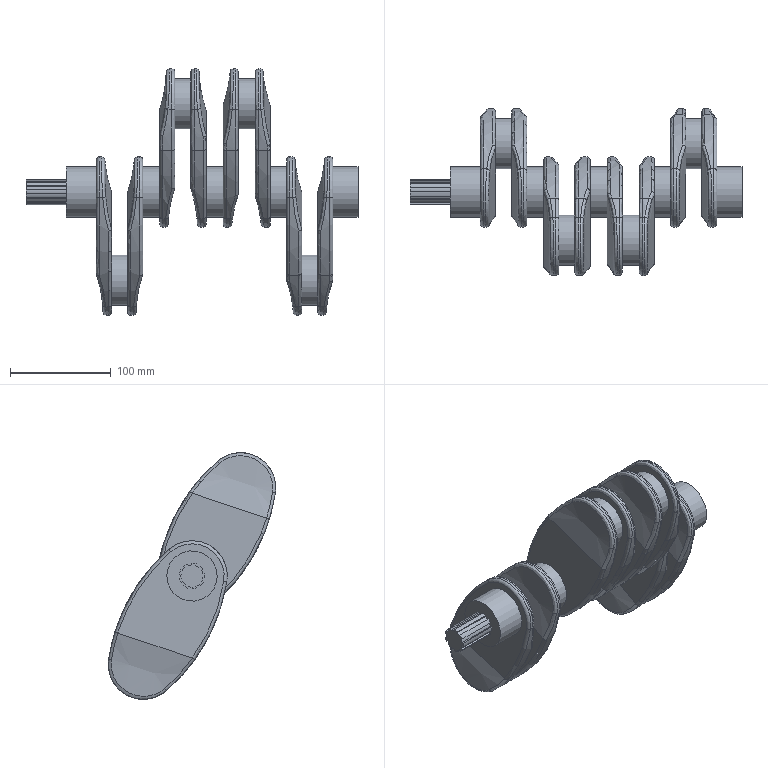Component | NX | CRANKSHAFT | 13 solids | 256 faces | volume 1556455 mm3 | spline 94 | cylinder 53 | plane 49 | torus 42 | other 18 | commonest cylinder face diameters 362.38 x16 70 x10 50 x9 25.4 x9 22 x9